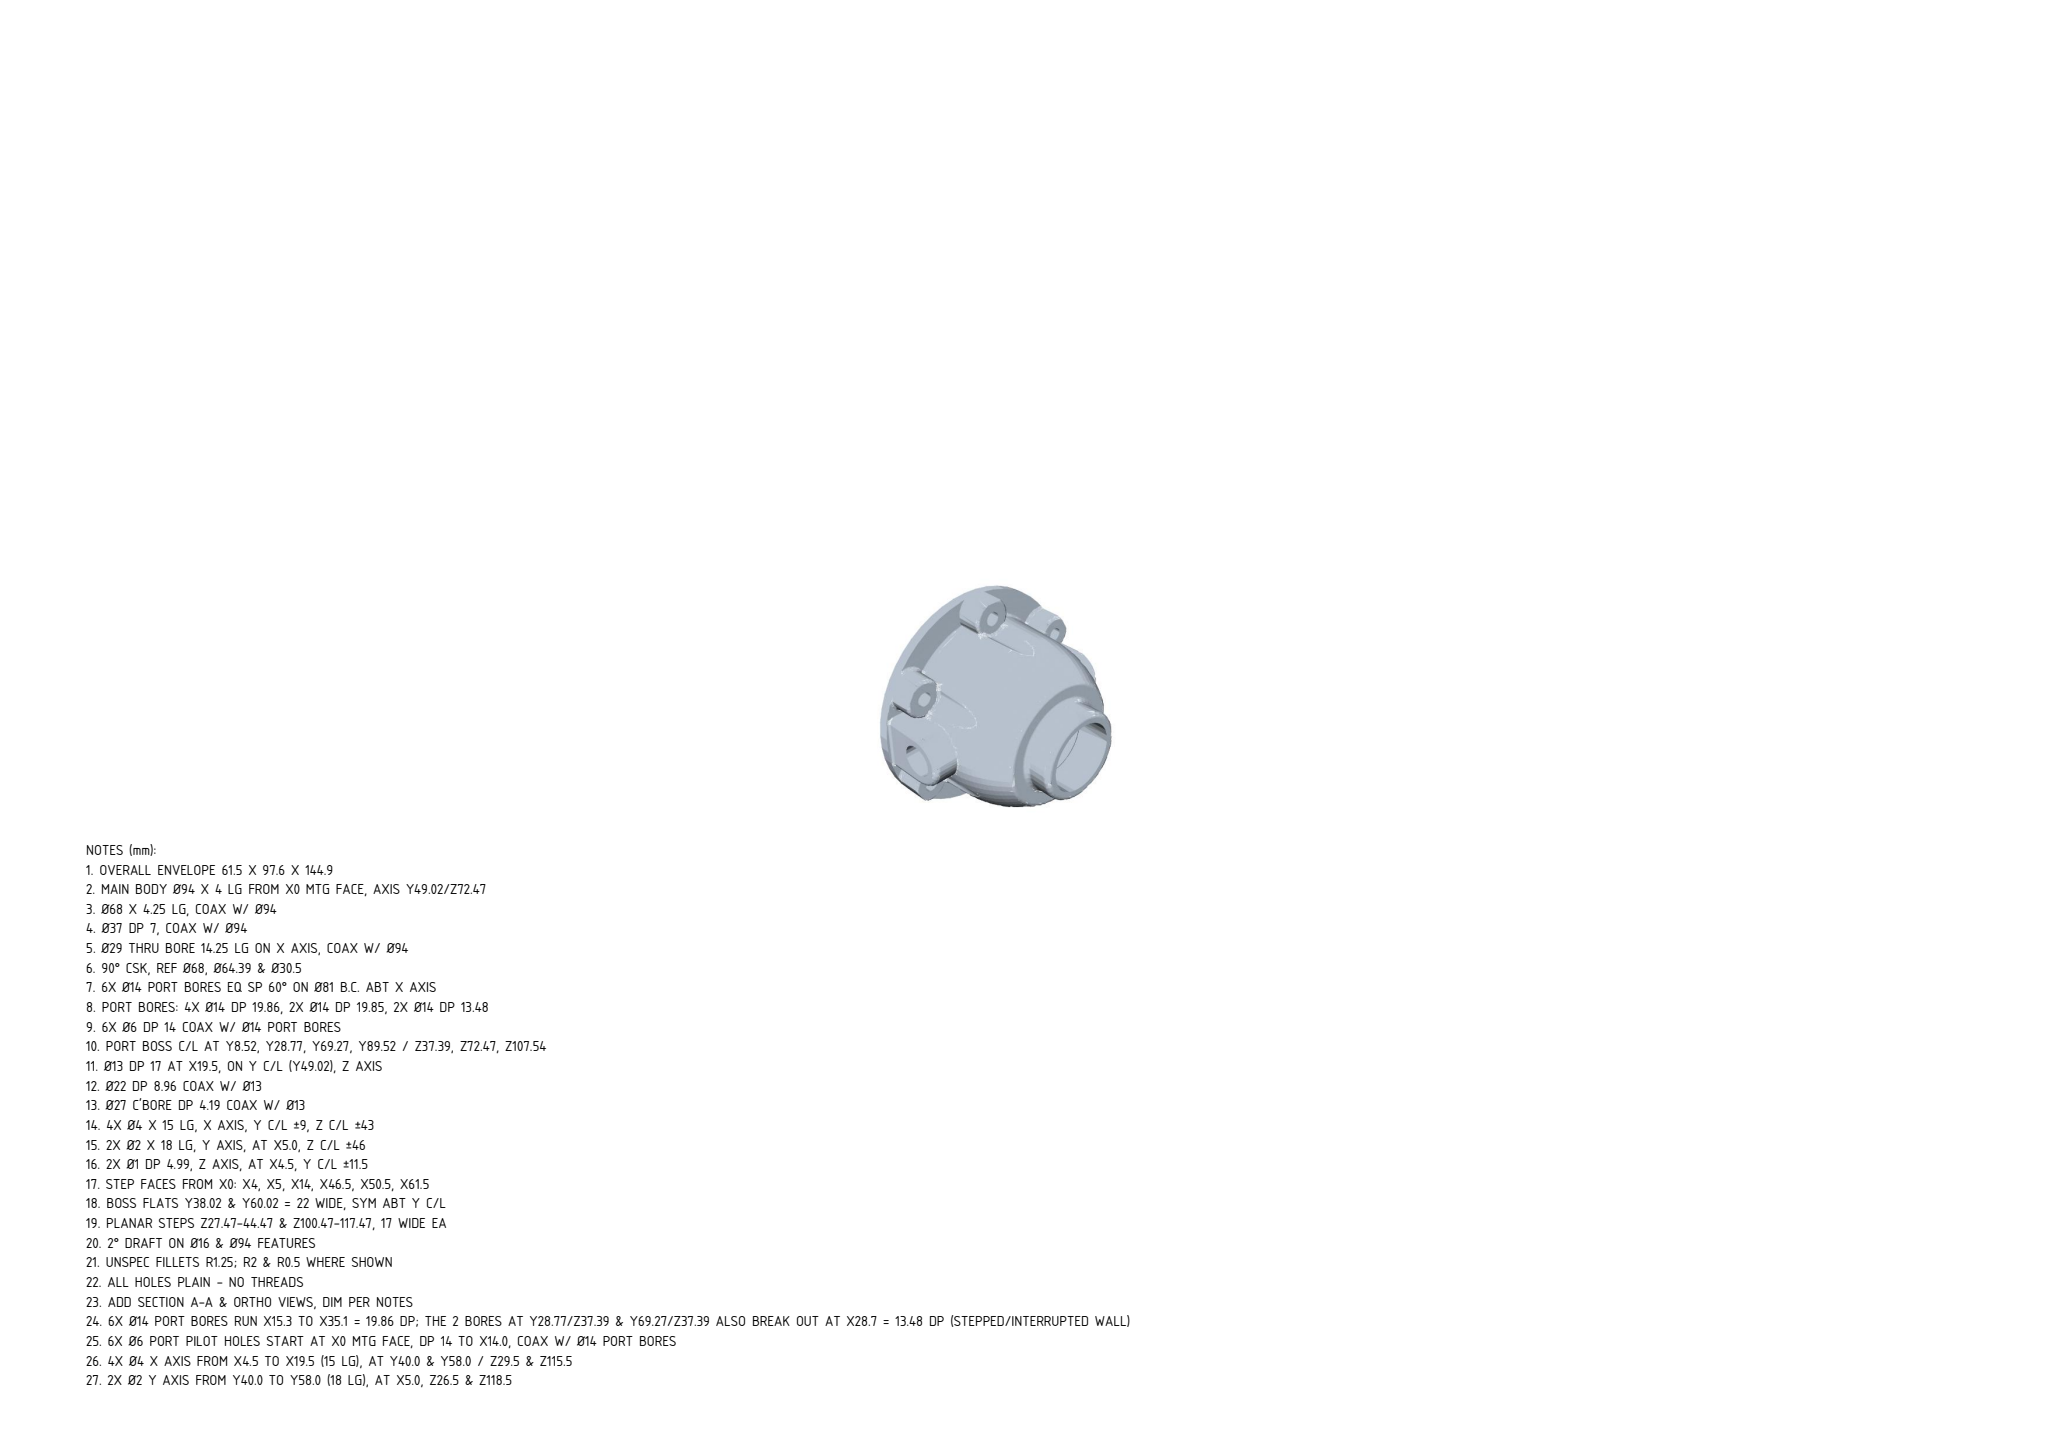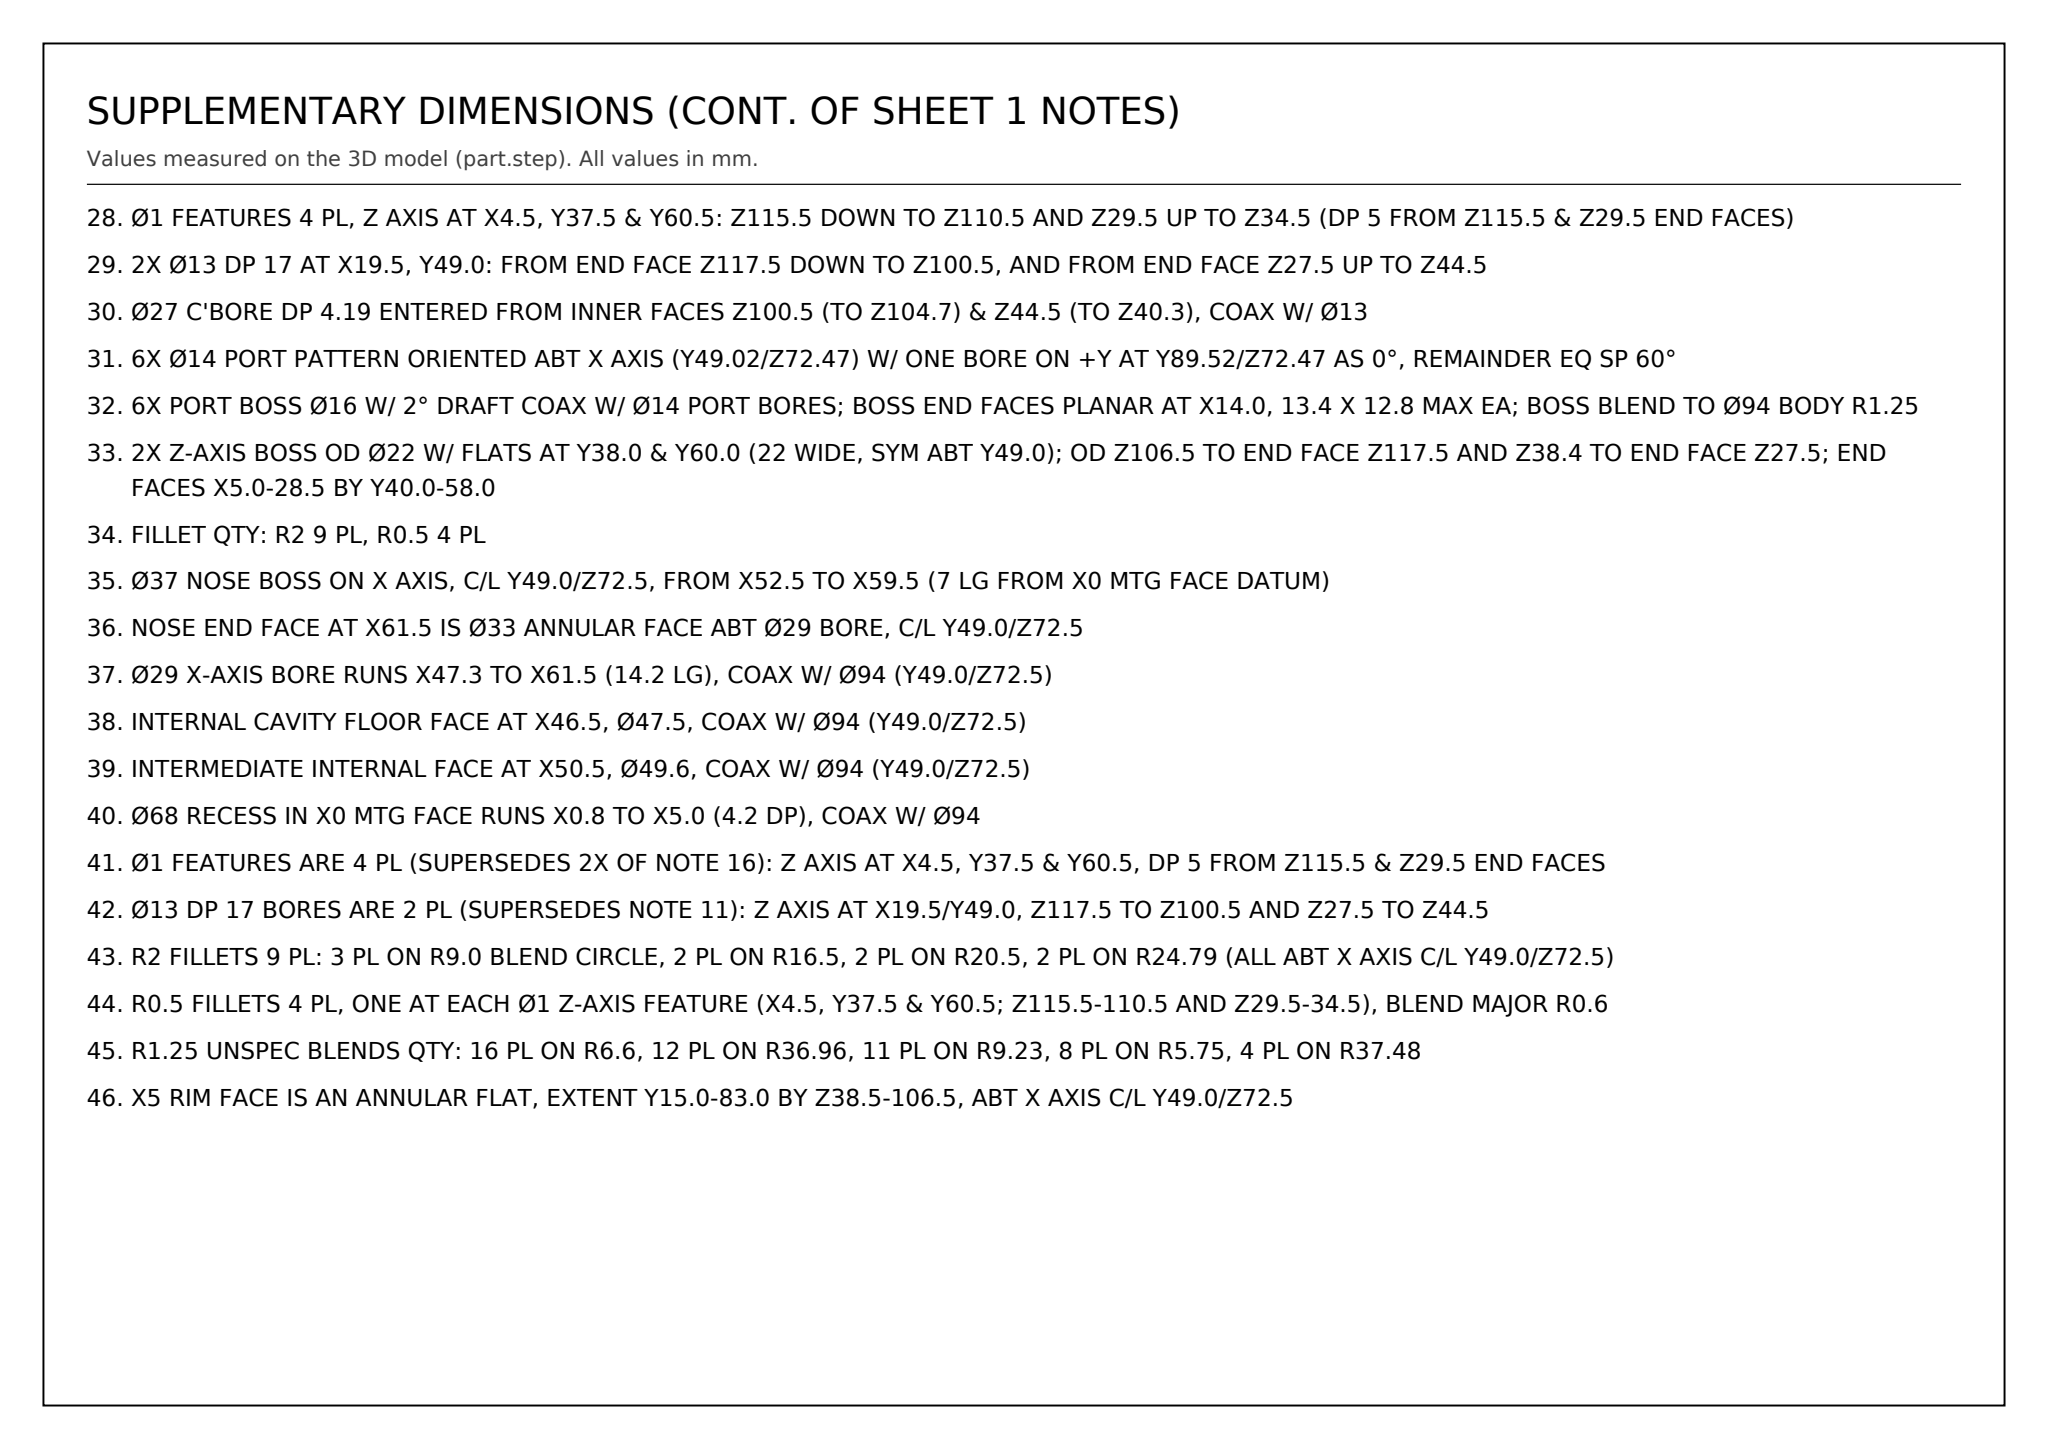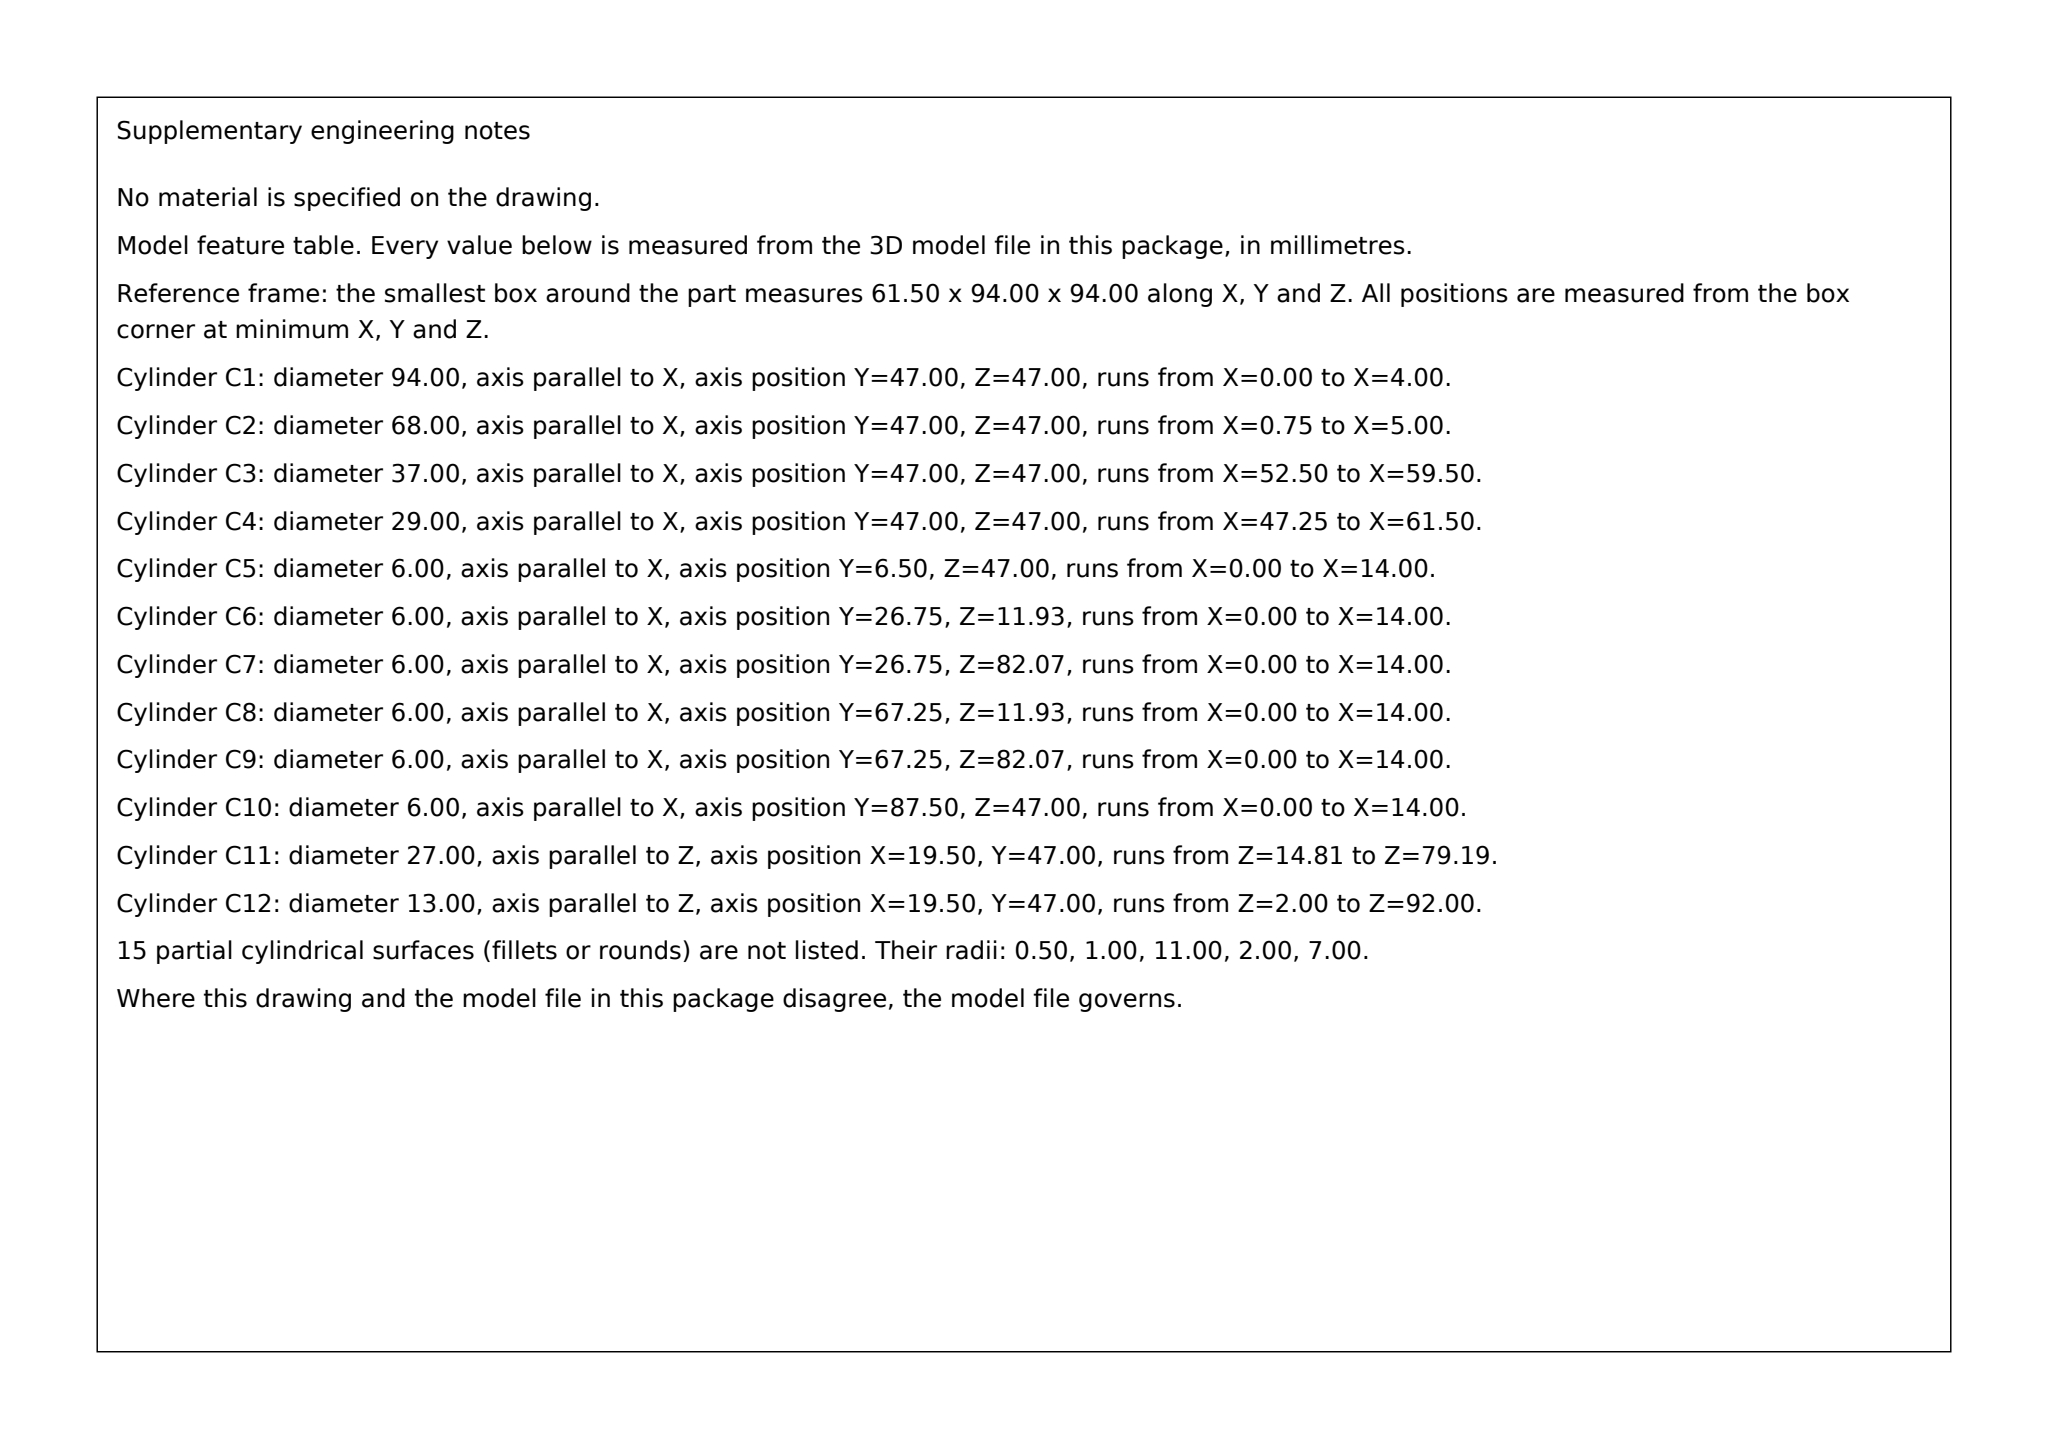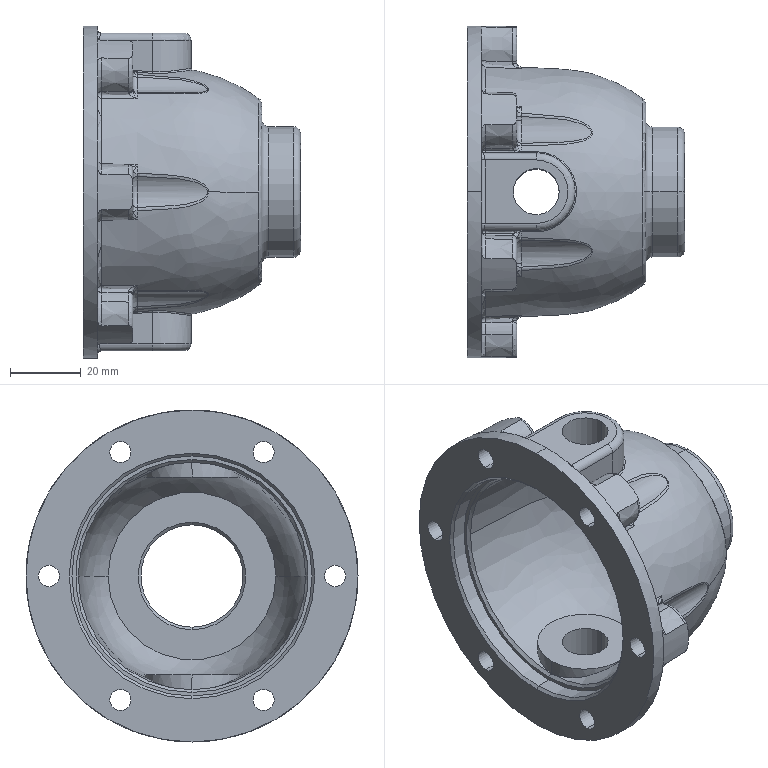Part | SolidWorks | mm | 1 solid | 274 faces | box 61.5 x 94 x 94 mm | volume 74433 mm3 | spline 96 | torus 64 | cylinder 49 | cone 30 | plane 25 | sphere 10 | commonest cylinder face diameters 6 x12 14 x8 13 x4 27 x4 1 x4 4 x4 22 x3 68 x2
Drawing notes:
OVERALL ENVELOPE 61.5 X 97.6 X 144.9 | from the solid: bbox_xyz [61.5, 97.612, 144.935]
MAIN BODY Ø94 X 4 LG FROM X0 MTG FACE, AXIS Y49.02/Z72.47 | from the solid: cyl 94 dia, x axis, pos [49.02,72.47], len 4; planes x0, x4
Ø68 X 4.25 LG, COAX W/ Ø94 | from the solid: cyl 68 dia, x axis, pos [49.02,72.47], len 4.25
Ø37 DP 7, COAX W/ Ø94 | from the solid: cyl 37 dia, x axis, pos [49.02,72.47], len 7
Ø29 THRU BORE 14.25 LG ON X AXIS, COAX W/ Ø94 | from the solid: cyl 29 dia, x axis, pos [49.02,72.47], len 14.25
90° CSK, REF Ø68, Ø64.39 & Ø30.5 | from the solid: cones [90,68], [90,64.393], [90,30.5]
6X Ø14 PORT BORES EQ SP 60° ON Ø81 B.C. ABT X AXIS | from the solid: Ø14 bores at R=40.5 from axis Y49.02/Z72.47, 6 places
PORT BORES: 4X Ø14 DP 19.86, 2X Ø14 DP 19.85, 2X Ø14 DP 13.48 | from the solid: cyl 14 len 19.86 x4, 19.85 x2, 13.48 x2
6X Ø6 DP 14 COAX W/ Ø14 PORT BORES | from the solid: cyl 6 dia, x axis, 6 locations, len 14
PORT BOSS C/L AT Y8.52, Y28.77, Y69.27, Y89.52 / Z37.39, Z72.47, Z107.54 | from the solid: cyl 6/14 positions list
Ø13 DP 17 AT X19.5, ON Y C/L (Y49.02), Z AXIS | from the solid: cyl 13 dia, z axis, pos [19.5,49.02], len 17
Ø22 DP 8.96 COAX W/ Ø13 | from the solid: cyl 22 dia, z axis, pos [19.5,49.02], len 8.96
Ø27 C'BORE DP 4.19 COAX W/ Ø13 | from the solid: cyl 27 dia, z axis, pos [19.5,49.02], len 4.19
4X Ø4 X 15 LG, X AXIS, Y C/L ±9, Z C/L ±43 | from the solid: cyl 4 dia at Y40.02/58.02, Z29.47/115.47, len 15
2X Ø2 X 18 LG, Y AXIS, AT X5.0, Z C/L ±46 | from the solid: cyl 2 dia, y axis, [5.0,z26.47] & [5.0,z118.47], len 18
2X Ø1 DP 4.99, Z AXIS, AT X4.5, Y C/L ±11.5 | from the solid: cyl 1 dia, z axis, [4.5,37.52] & [4.5,60.52], len 4.99
STEP FACES FROM X0: X4, X5, X14, X46.5, X50.5, X61.5 | from the solid: axis_planes x = 0, 4, 5, 14, 46.5, 50.5, 61.5
BOSS FLATS Y38.02 & Y60.02 = 22 WIDE, SYM ABT Y C/L | from the solid: axis_planes y 38.02 & 60.02; axis Y49.02
PLANAR STEPS Z27.47-44.47 & Z100.47-117.47, 17 WIDE EA | from the solid: axis_planes z 27.47, 44.47, 100.47, 117.47
2° DRAFT ON Ø16 & Ø94 FEATURES | from the solid: cones [2,16] x18, [2,94] x6
UNSPEC FILLETS R1.25; R2 & R0.5 WHERE SHOWN | from the solid: fillet_radii [2,9],[1.25,51],[0.5,4]
ALL HOLES PLAIN - NO THREADS | from the solid: no thread/helix features in STEP cylinder list
ADD SECTION A-A & ORTHO VIEWS, DIM PER NOTES | from the solid: model pictorial only; all features defined by STEP coords
6X Ø14 PORT BORES RUN X15.3 TO X35.1 = 19.86 DP; THE 2 BORES AT Y28.77/Z37.39 & Y69.27/Z37.39 ALSO BREAK OUT AT X28.7 = 13.48 DP (STEPPED/INTERRUPTED WALL) | from the solid: cylinders: concave arc Ø14 x-axis from 15.3 to 35.1 at 6 y/z locations, plus 13.4-long Ø14 arcs at (y28.8,z37.4) and (y69.3,z37.4)
6X Ø6 PORT PILOT HOLES START AT X0 MTG FACE, DP 14 TO X14.0, COAX W/ Ø14 PORT BORES | from the solid: cylinders: hole/bore Ø6 x-axis from 0.0 to 14.0 at the six port y/z locations
4X Ø4 X AXIS FROM X4.5 TO X19.5 (15 LG), AT Y40.0 & Y58.0 / Z29.5 & Z115.5 | from the solid: cylinders: convex arc Ø4 x-axis from 4.5 to 19.5 at (y40,z115.5),(y40,z29.5),(y58,z115.5),(y58,z29.5)
2X Ø2 Y AXIS FROM Y40.0 TO Y58.0 (18 LG), AT X5.0, Z26.5 & Z118.5 | from the solid: cylinders: concave arc Ø2 y-axis from 40.0 to 58.0 at (x5.0,z118.5) and (x5.0,z26.5)
Ø1 FEATURES 4 PL, Z AXIS AT X4.5, Y37.5 & Y60.5: Z115.5 DOWN TO Z110.5 AND Z29.5 UP TO Z34.5 (DP 5 FROM Z115.5 & Z29.5 END FACES) | from the solid: cylinders: concave arc Ø1 z-axis 110.5-115.5 and 29.5-34.5 at (4.5,37.5) and (4.5,60.5)
2X Ø13 DP 17 AT X19.5, Y49.0: FROM END FACE Z117.5 DOWN TO Z100.5, AND FROM END FACE Z27.5 UP TO Z44.5 | from the solid: cylinders: hole/bore Ø13 z-axis at (19.5,49.0) from 100.5 to 117.5 and from 27.5 to 44.5
Ø27 C'BORE DP 4.19 ENTERED FROM INNER FACES Z100.5 (TO Z104.7) & Z44.5 (TO Z40.3), COAX W/ Ø13 | from the solid: cylinders: Ø27 z-axis at (19.5,49.0) from 100.5 to 104.7 and from 40.3 to 44.5; planar faces z=100.5 and z=44.5
6X Ø14 PORT PATTERN ORIENTED ABT X AXIS (Y49.02/Z72.47) W/ ONE BORE ON +Y AT Y89.52/Z72.47 AS 0°, REMAINDER EQ SP 60° | from the solid: port bore axis positions (y,z): (89.5,72.5),(69.3,107.5),(28.8,107.5),(8.5,72.5),(28.8,37.4),(69.3,37.4) on R40.5 about (49.0,72.5)
6X PORT BOSS Ø16 W/ 2° DRAFT COAX W/ Ø14 PORT BORES; BOSS END FACES PLANAR AT X14.0, 13.4 X 12.8 MAX EA; BOSS BLEND TO Ø94 BODY R1.25 | from the solid: cones included angle 2°, ref dia 16 (15 PL); axis_planes x=14.0 (6 faces, area 99 ea); tori minor_r 1.25
2X Z-AXIS BOSS OD Ø22 W/ FLATS AT Y38.0 & Y60.0 (22 WIDE, SYM ABT Y49.0); OD Z106.5 TO END FACE Z117.5 AND Z38.4 TO END FACE Z27.5; END FACES X5.0-28.5 BY Y40.0-58.0 | from the solid: cylinders: convex arc Ø22 z-axis 106.5-115.5 & 29.5-38.4 at (19.5,49.0); planes y=38.0/y=60.0 x[4.5,19.5]; planes z=117.5 & z=27.5 x[5.0,28.5] y[40.0,58.0]
FILLET QTY: R2 9 PL, R0.5 4 PL | from the solid: tori: minor_r 2.0 (major 9.0 x3, 16.5 x2, 20.5 x2, 24.79 x2 = 9); minor_r 0.5 x4
Ø37 NOSE BOSS ON X AXIS, C/L Y49.0/Z72.5, FROM X52.5 TO X59.5 (7 LG FROM X0 MTG FACE DATUM) | from the solid: cylinders: boss/shaft Ø37.0 axis x at (y49.0,z72.5) from 52.5 to 59.5
NOSE END FACE AT X61.5 IS Ø33 ANNULAR FACE ABT Ø29 BORE, C/L Y49.0/Z72.5 | from the solid: axis_planes: normal x, offset 61.5, extent y[32.5,65.5] z[56.0,89.0] (33.0 across, centered 49.0/72.5)
Ø29 X-AXIS BORE RUNS X47.3 TO X61.5 (14.2 LG), COAX W/ Ø94 (Y49.0/Z72.5) | from the solid: cylinders: hole/bore Ø29.0 axis x at (y49.0,z72.5) from 47.3 to 61.5
INTERNAL CAVITY FLOOR FACE AT X46.5, Ø47.5, COAX W/ Ø94 (Y49.0/Z72.5) | from the solid: axis_planes: normal x, offset 46.5, extent y[25.3,72.8] z[48.7,96.2] (47.5 across, centered 49.0/72.5)
INTERMEDIATE INTERNAL FACE AT X50.5, Ø49.6, COAX W/ Ø94 (Y49.0/Z72.5) | from the solid: axis_planes: normal x, offset 50.5, extent y[24.2,73.8] z[47.7,97.3] (49.6 across, centered 49.0/72.5)
Ø68 RECESS IN X0 MTG FACE RUNS X0.8 TO X5.0 (4.2 DP), COAX W/ Ø94 | from the solid: cylinders: hole/bore Ø68.0 axis x at (y49.0,z72.5) from 0.8 to 5.0
Ø1 FEATURES ARE 4 PL (SUPERSEDES 2X OF NOTE 16): Z AXIS AT X4.5, Y37.5 & Y60.5, DP 5 FROM Z115.5 & Z29.5 END FACES | from the solid: cylinders: four Ø1.0 z-axis arcs at (4.5,37.5) and (4.5,60.5), 110.5-115.5 and 29.5-34.5
Ø13 DP 17 BORES ARE 2 PL (SUPERSEDES NOTE 11): Z AXIS AT X19.5/Y49.0, Z117.5 TO Z100.5 AND Z27.5 TO Z44.5 | from the solid: cylinders: two hole/bore Ø13.0 z-axis at (19.5,49.0), 100.5-117.5 and 27.5-44.5
R2 FILLETS 9 PL: 3 PL ON R9.0 BLEND CIRCLE, 2 PL ON R16.5, 2 PL ON R20.5, 2 PL ON R24.79 (ALL ABT X AXIS C/L Y49.0/Z72.5) | from the solid: tori[minor_r,major_r]: [2.0, major 9.0, 3], [2.0, major 16.5, 2], [2.0, major 20.5, 2], [2.0, major 24.79, 2]
R0.5 FILLETS 4 PL, ONE AT EACH Ø1 Z-AXIS FEATURE (X4.5, Y37.5 & Y60.5; Z115.5-110.5 AND Z29.5-34.5), BLEND MAJOR R0.6 | from the solid: tori [0.5, major 0.6, 4] and Ø1 90° arcs at z axis [4.5,37.5] and [4.5,60.5], from 110.5-115.5 / 29.5-34.5
R1.25 UNSPEC BLENDS QTY: 16 PL ON R6.6, 12 PL ON R36.96, 11 PL ON R9.23, 8 PL ON R5.75, 4 PL ON R37.48 | from the solid: tori [1.25, major 6.6, 16], [1.25, major 36.96, 12], [1.25, major 9.23, 11], [1.25, major 5.75, 8], [1.25, major 37.48, 4]
X5 RIM FACE IS AN ANNULAR FLAT, EXTENT Y15.0-83.0 BY Z38.5-106.5, ABT X AXIS C/L Y49.0/Z72.5 | from the solid: axis_planes x 5.0 extent {'y': [15.0, 83.0], 'z': [38.5, 106.5]} area 213